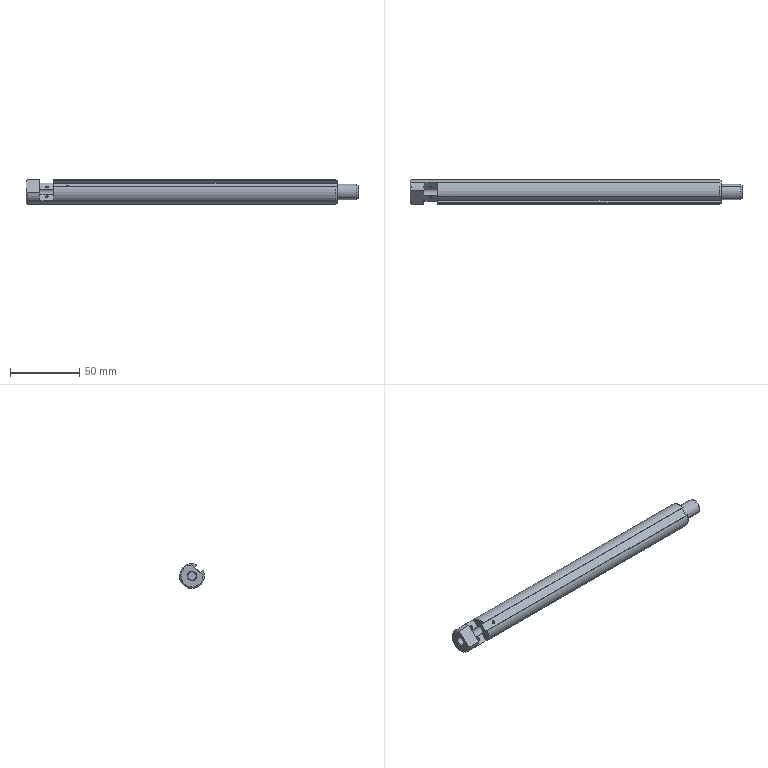Component | SolidWorks | JJDJR-3060-E-004-1 | 1 solid | 46 faces | volume 51816 mm3 | cylinder 18 | cone 14 | plane 14 | commonest cylinder face diameters 18 x5 2.05 x4 6 x3 2 x2 5 x2 11 x2 | material 40Cr